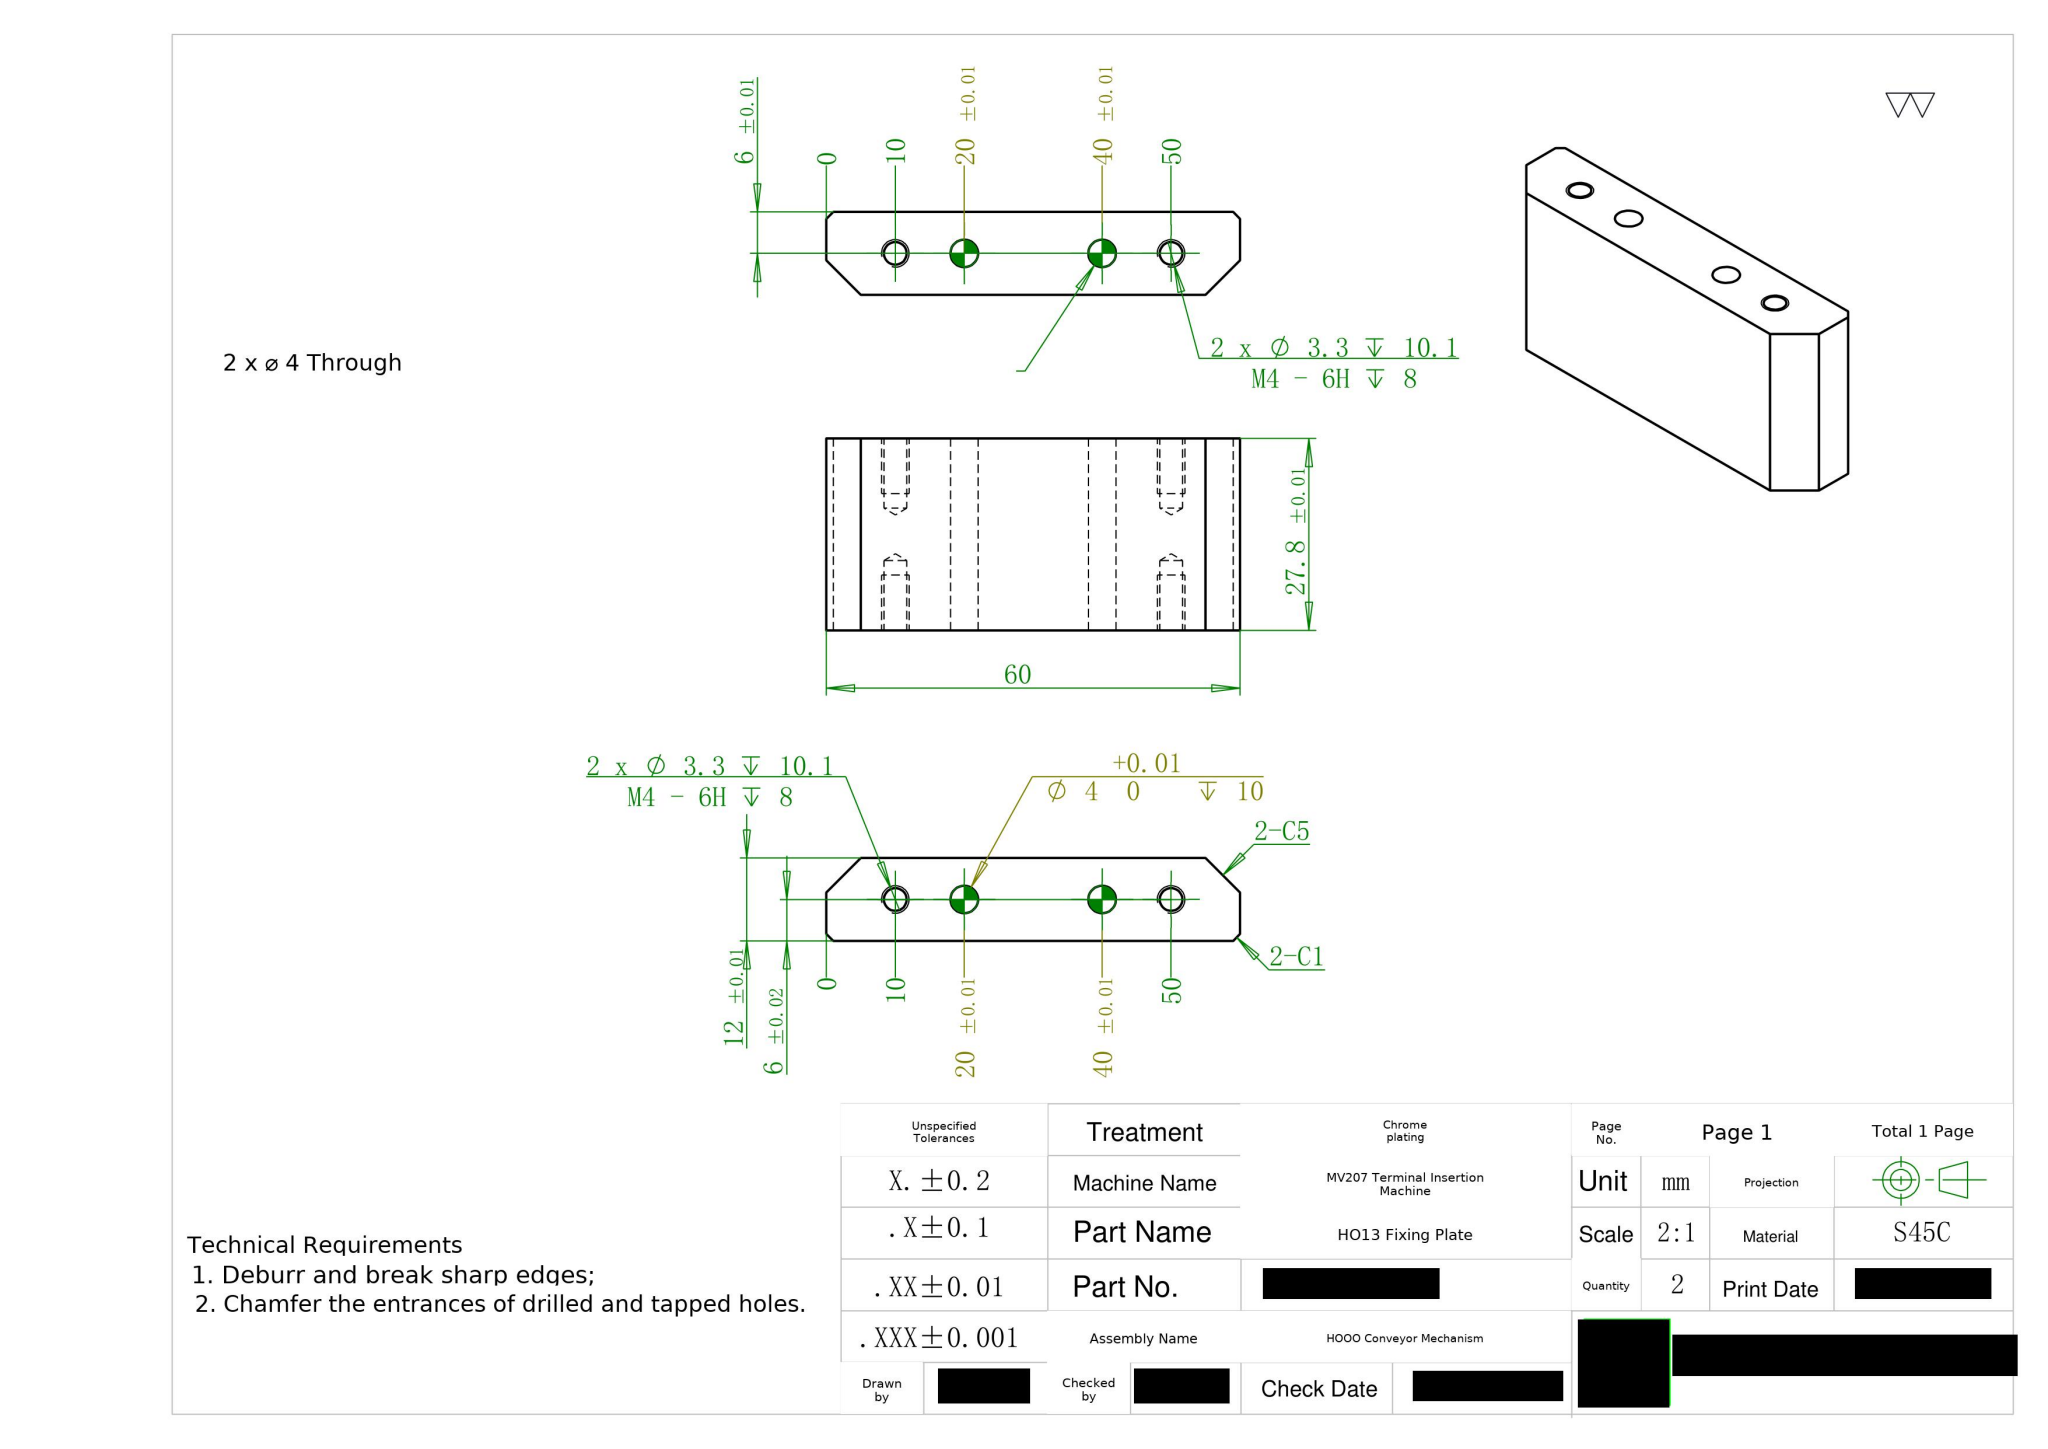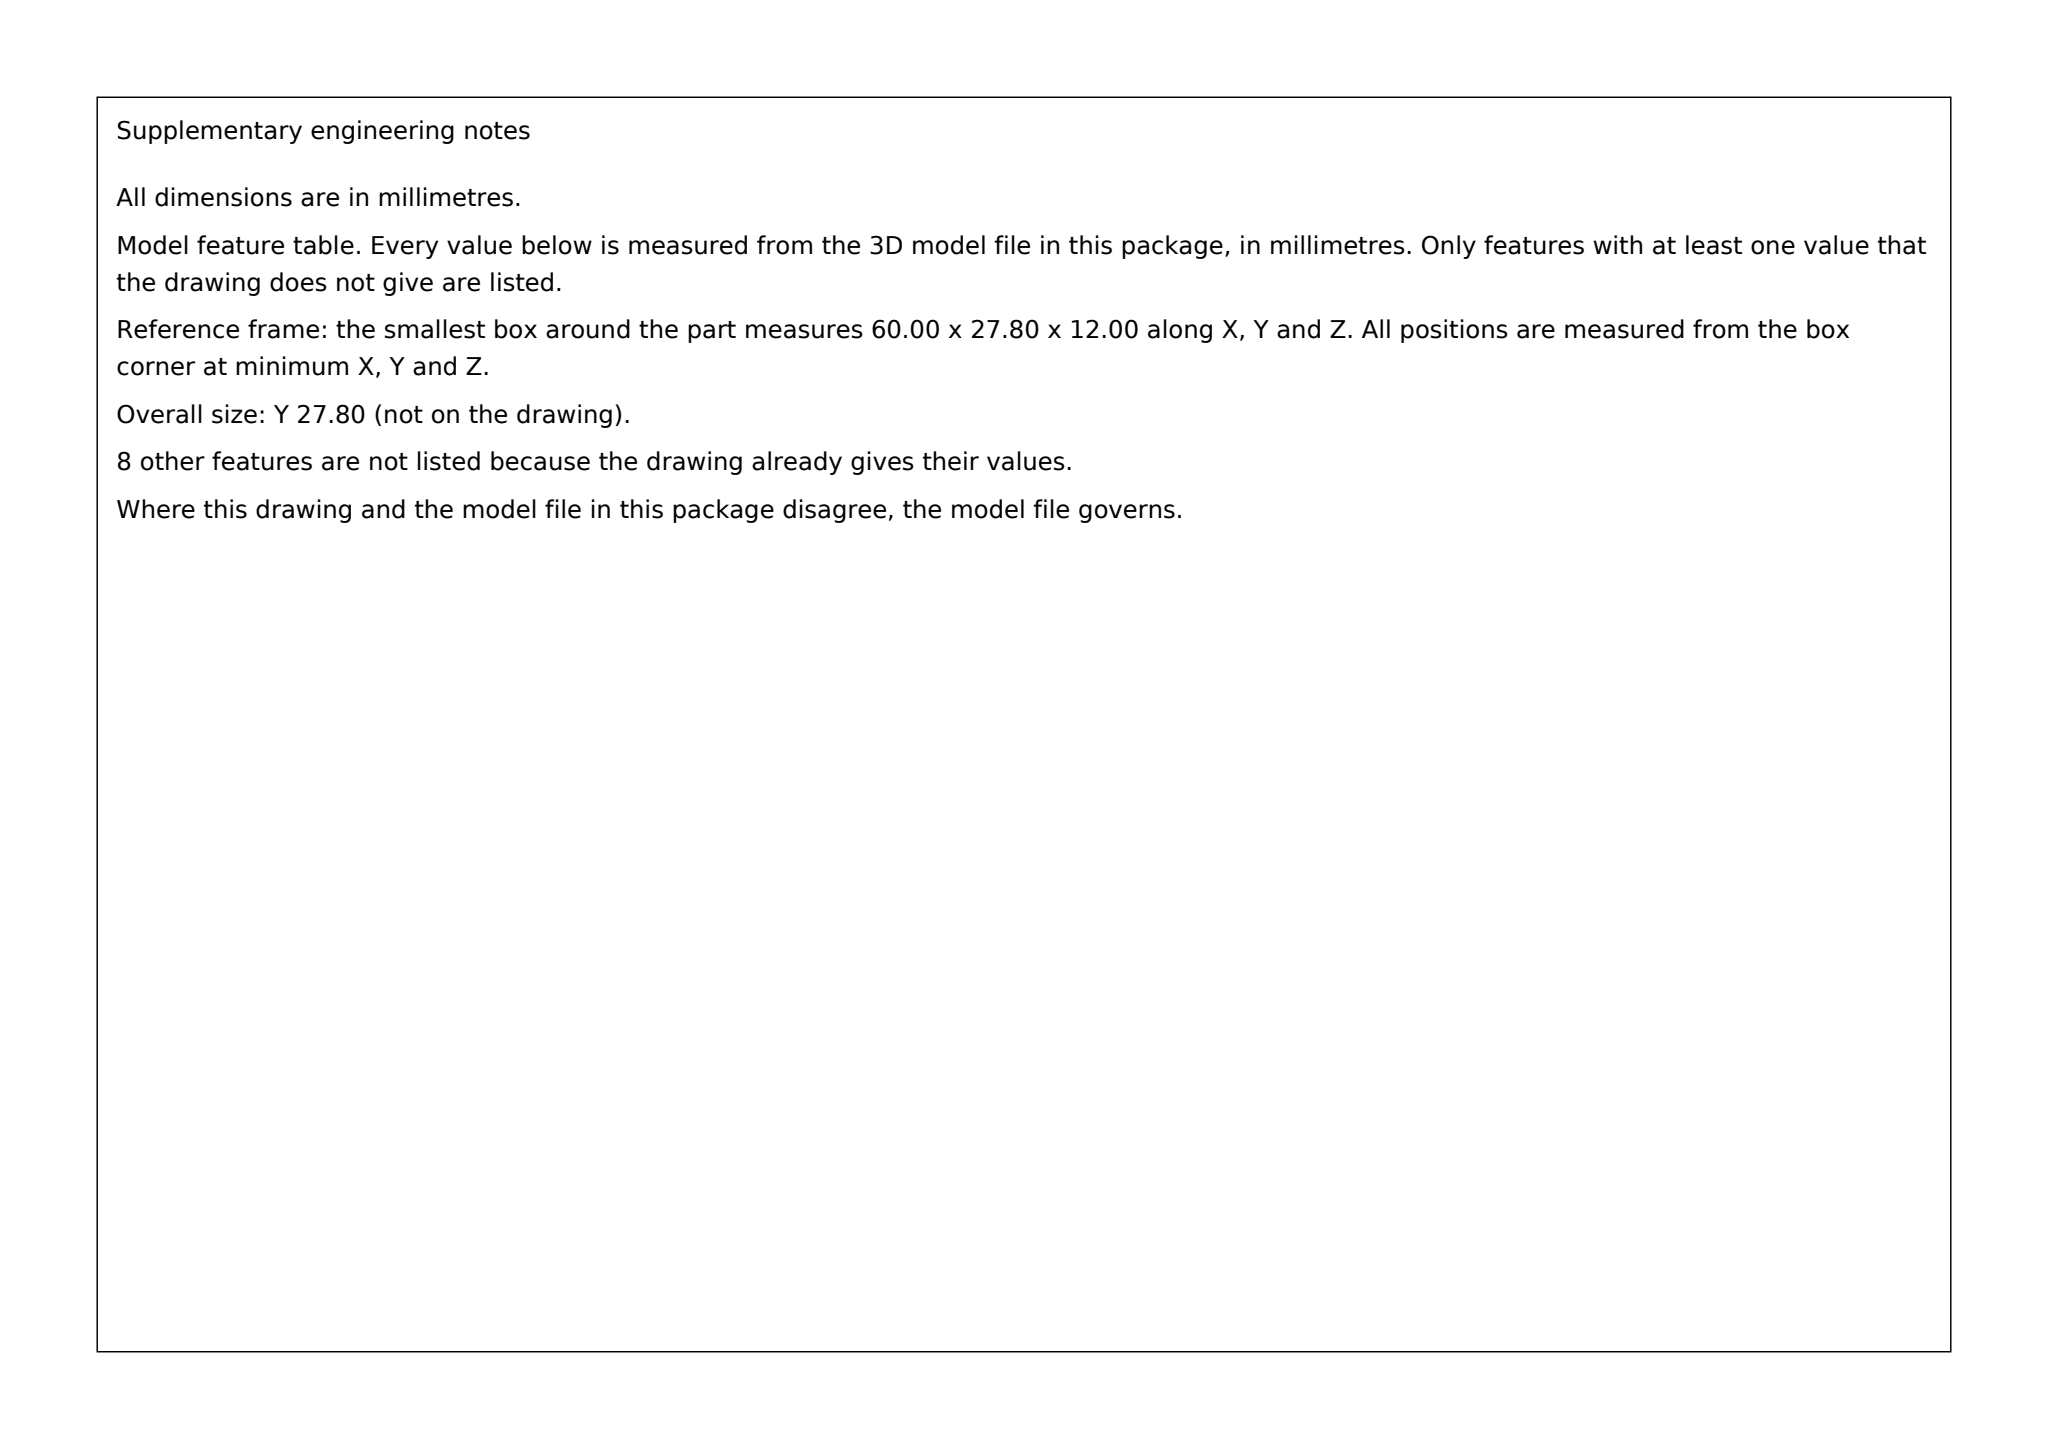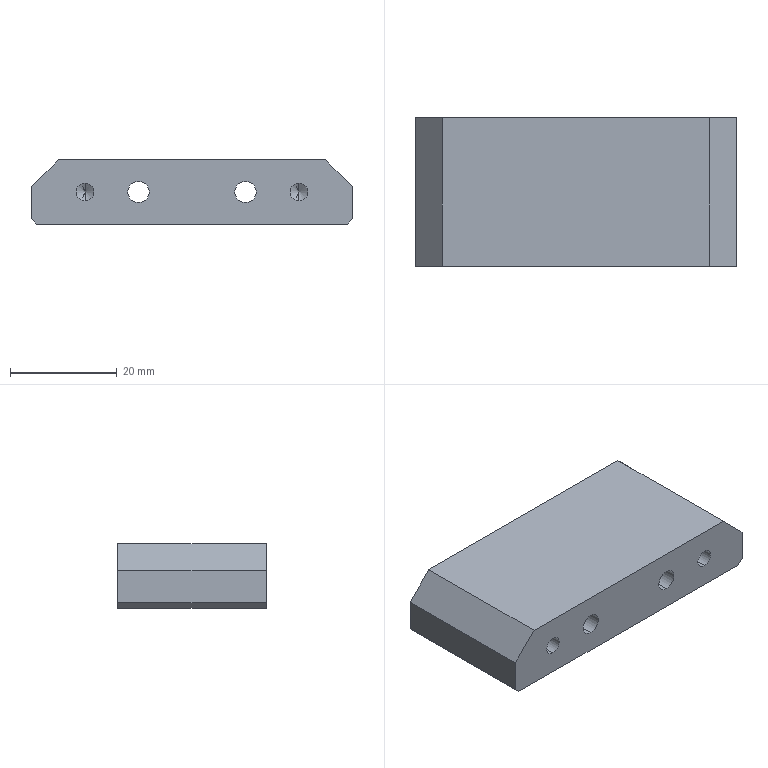Part | SolidWorks | mm | material S45C | 1 solid | 30 faces | box 60 x 27.8 x 12 mm | volume 18238 mm3 | cylinder 12 | plane 10 | cone 8 | commonest cylinder face diameters 3.3 x8 4 x4
build123d program:
from build123d import *

# Parameters (mm, degrees)
SKETCH1_W                    = 60
SKETCH1_H                    = 27.8
BOSS_EXTRUDE1_DEPTH          = 12
M4_TAPPED_HOLE1_D            = 3.3
M4_TAPPED_HOLE1_DEPTH        = 10.1
M4_TAPPED_HOLE1_TIP          = 0.9914
M4_TAPPED_HOLE2_D            = 3.3
M4_TAPPED_HOLE2_DEPTH        = 10.1
M4_TAPPED_HOLE2_TIP          = 0.9914
CHAMFER1_SIZE                = 5
F_4_0_4_DIAMETER_HOLE1_D     = 4
F_4_0_4_DIAMETER_HOLE2_D     = 4
F_4_0_4_DIAMETER_HOLE2_DEPTH = 10
F_4_0_4_DIAMETER_HOLE2_TIP   = 1.202
CHAMFER2_SIZE                = 1


with BuildPart() as part:
    # Sketch1 → Boss-Extrude1 (new body)
    with BuildSketch(Plane.XY):
        Rectangle(SKETCH1_W, SKETCH1_H)
    extrude(amount=BOSS_EXTRUDE1_DEPTH)

    # M4 Tapped Hole1
    with Locations(Plane(origin=(0, 13.9, 0), x_dir=(1, 0, 0), z_dir=(0, 1, 0))):
        with Locations((-20, -6), (20, -6)):
            Hole(M4_TAPPED_HOLE1_D / 2, depth=M4_TAPPED_HOLE1_DEPTH)
            with Locations((0, 0, -(M4_TAPPED_HOLE1_DEPTH + M4_TAPPED_HOLE1_TIP / 2))):  # 118° drill point
                Cone(0, M4_TAPPED_HOLE1_D / 2, M4_TAPPED_HOLE1_TIP, mode=Mode.SUBTRACT)

    # M4 Tapped Hole2
    with Locations(Plane(origin=(0, -13.9, 0), x_dir=(-1, 0, 0), z_dir=(0, -1, 0))):
        with Locations((20, -6), (-20, -6)):
            Hole(M4_TAPPED_HOLE2_D / 2, depth=M4_TAPPED_HOLE2_DEPTH)
            with Locations((0, 0, -(M4_TAPPED_HOLE2_DEPTH + M4_TAPPED_HOLE2_TIP / 2))):  # 118° drill point
                Cone(0, M4_TAPPED_HOLE2_D / 2, M4_TAPPED_HOLE2_TIP, mode=Mode.SUBTRACT)

    # Chamfer1
    chamfer1_edges = [part.edges().sort_by_distance(p)[0] for p in [
        (-30, 0, 12),
        (30, 0, 12),
    ]]
    chamfer(chamfer1_edges, length=CHAMFER1_SIZE)

    # 4.0 _4_ Diameter Hole1 (through all)
    with Locations(Plane(origin=(0, 13.9, 0), x_dir=(1, 0, 0), z_dir=(0, 1, 0))):
        with Locations((-10, -6), (10, -6)):
            Hole(F_4_0_4_DIAMETER_HOLE1_D / 2)

    # 4.0 _4_ Diameter Hole2
    with Locations(Plane(origin=(0, -13.9, 0), x_dir=(-1, 0, 0), z_dir=(0, -1, 0))):
        with Locations((10, -6), (-10, -6)):
            Hole(F_4_0_4_DIAMETER_HOLE2_D / 2, depth=F_4_0_4_DIAMETER_HOLE2_DEPTH)
            with Locations((0, 0, -(F_4_0_4_DIAMETER_HOLE2_DEPTH + F_4_0_4_DIAMETER_HOLE2_TIP / 2))):  # 118° drill point
                Cone(0, F_4_0_4_DIAMETER_HOLE2_D / 2, F_4_0_4_DIAMETER_HOLE2_TIP, mode=Mode.SUBTRACT)

    # Chamfer2
    chamfer2_edges = [part.edges().sort_by_distance(p)[0] for p in [
        (-30, 0, 0),
        (30, 0, 0),
    ]]
    chamfer(chamfer2_edges, length=CHAMFER2_SIZE)


solid = part.part
STEP:
#1=CARTESIAN_POINT('',(-10.,-13.9,4.));
#2=VERTEX_POINT('',#1);
#3=CARTESIAN_POINT('',(-10.,-13.9,8.));
#4=VERTEX_POINT('',#3);
#5=CARTESIAN_POINT('',(-10.,-13.9,6.));
#6=DIRECTION('',(0.,1.,0.));
#7=DIRECTION('',(0.,0.,1.));
#8=AXIS2_PLACEMENT_3D('',#5,#6,#7);
#9=CIRCLE('',#8,2.);
#10=EDGE_CURVE('',#2,#4,#9,.T.);
#11=ORIENTED_EDGE('',*,*,#10,.F.);
#12=CARTESIAN_POINT('',(-10.,13.9,4.));
#13=VERTEX_POINT('',#12);
#14=CARTESIAN_POINT('',(-10.,13.9,4.));
#15=DIRECTION('',(0.,1.,0.));
#16=VECTOR('',#15,1000.);
#17=LINE('',#14,#16);
#18=EDGE_CURVE('',#2,#13,#17,.T.);
#19=ORIENTED_EDGE('',*,*,#18,.T.);
#20=CARTESIAN_POINT('',(-10.,13.9,8.));
#21=VERTEX_POINT('',#20);
#22=CARTESIAN_POINT('',(-10.,13.9,6.));
#23=DIRECTION('',(0.,1.,0.));
#24=DIRECTION('',(0.,0.,1.));
#25=AXIS2_PLACEMENT_3D('',#22,#23,#24);
#26=CIRCLE('',#25,2.);
#27=EDGE_CURVE('',#13,#21,#26,.T.);
#28=ORIENTED_EDGE('',*,*,#27,.T.);
#29=CARTESIAN_POINT('',(-10.,13.9,8.));
#30=DIRECTION('',(0.,1.,0.));
#31=VECTOR('',#30,1000.);
#32=LINE('',#29,#31);
#33=EDGE_CURVE('',#4,#21,#32,.T.);
#34=ORIENTED_EDGE('',*,*,#33,.F.);
#35=EDGE_LOOP('',(#11,#19,#28,#34));
#36=FACE_OUTER_BOUND('',#35,.T.);
#37=CARTESIAN_POINT('',(-10.,13.9,6.));
#38=DIRECTION('',(0.,1.,0.));
#39=DIRECTION('',(0.,0.,1.));
#40=AXIS2_PLACEMENT_3D('',#37,#38,#39);
#41=CYLINDRICAL_SURFACE('',#40,2.);
#42=ADVANCED_FACE('',(#36),#41,.F.);
#43=CARTESIAN_POINT('',(10.,-13.9,4.));
#44=VERTEX_POINT('',#43);
#45=CARTESIAN_POINT('',(10.,-13.9,8.));
#46=VERTEX_POINT('',#45);
#47=CARTESIAN_POINT('',(10.,-13.9,6.));
#48=DIRECTION('',(0.,1.,0.));
#49=DIRECTION('',(0.,0.,1.));
#50=AXIS2_PLACEMENT_3D('',#47,#48,#49);
#51=CIRCLE('',#50,2.);
#52=EDGE_CURVE('',#44,#46,#51,.T.);
#53=ORIENTED_EDGE('',*,*,#52,.F.);
#54=CARTESIAN_POINT('',(10.,13.9,4.));
#55=VERTEX_POINT('',#54);
#56=CARTESIAN_POINT('',(10.,13.9,4.));
#57=DIRECTION('',(0.,1.,0.));
#58=VECTOR('',#57,1000.);
#59=LINE('',#56,#58);
#60=EDGE_CURVE('',#44,#55,#59,.T.);
#61=ORIENTED_EDGE('',*,*,#60,.T.);
#62=CARTESIAN_POINT('',(10.,13.9,8.));
#63=VERTEX_POINT('',#62);
#64=CARTESIAN_POINT('',(10.,13.9,6.));
#65=DIRECTION('',(0.,1.,0.));
#66=DIRECTION('',(0.,0.,1.));
#67=AXIS2_PLACEMENT_3D('',#64,#65,#66);
#68=CIRCLE('',#67,2.);
#69=EDGE_CURVE('',#55,#63,#68,.T.);
#70=ORIENTED_EDGE('',*,*,#69,.T.);
#71=CARTESIAN_POINT('',(10.,13.9,8.));
#72=DIRECTION('',(0.,1.,0.));
#73=VECTOR('',#72,1000.);
#74=LINE('',#71,#73);
#75=EDGE_CURVE('',#46,#63,#74,.T.);
#76=ORIENTED_EDGE('',*,*,#75,.F.);
#77=EDGE_LOOP('',(#53,#61,#70,#76));
#78=FACE_OUTER_BOUND('',#77,.T.);
#79=CARTESIAN_POINT('',(10.,13.9,6.));
#80=DIRECTION('',(0.,1.,0.));
#81=DIRECTION('',(0.,0.,1.));
#82=AXIS2_PLACEMENT_3D('',#79,#80,#81);
#83=CYLINDRICAL_SURFACE('',#82,2.);
#84=ADVANCED_FACE('',(#78),#83,.F.);
#85=CARTESIAN_POINT('',(-20.,-3.8,7.65));
#86=VERTEX_POINT('',#85);
#87=CARTESIAN_POINT('',(-20.,-3.8,4.35));
#88=VERTEX_POINT('',#87);
#89=CARTESIAN_POINT('',(-20.,-3.8,6.));
#90=DIRECTION('',(0.,-1.,0.));
#91=DIRECTION('',(0.,0.,-1.));
#92=AXIS2_PLACEMENT_3D('',#89,#90,#91);
#93=CIRCLE('',#92,1.65);
#94=EDGE_CURVE('',#86,#88,#93,.T.);
#95=ORIENTED_EDGE('',*,*,#94,.F.);
#96=CARTESIAN_POINT('',(-20.,-13.9,7.65));
#97=VERTEX_POINT('',#96);
#98=CARTESIAN_POINT('',(-20.,-13.9,7.65));
#99=DIRECTION('',(0.,-1.,0.));
#100=VECTOR('',#99,1000.);
#101=LINE('',#98,#100);
#102=EDGE_CURVE('',#86,#97,#101,.T.);
#103=ORIENTED_EDGE('',*,*,#102,.T.);
#104=CARTESIAN_POINT('',(-20.,-13.9,4.35));
#105=VERTEX_POINT('',#104);
#106=CARTESIAN_POINT('',(-20.,-13.9,6.));
#107=DIRECTION('',(0.,-1.,0.));
#108=DIRECTION('',(0.,0.,-1.));
#109=AXIS2_PLACEMENT_3D('',#106,#107,#108);
#110=CIRCLE('',#109,1.65);
#111=EDGE_CURVE('',#97,#105,#110,.T.);
#112=ORIENTED_EDGE('',*,*,#111,.T.);
#113=CARTESIAN_POINT('',(-20.,-13.9,4.35));
#114=DIRECTION('',(0.,-1.,0.));
#115=VECTOR('',#114,1000.);
#116=LINE('',#113,#115);
#117=EDGE_CURVE('',#88,#105,#116,.T.);
#118=ORIENTED_EDGE('',*,*,#117,.F.);
#119=EDGE_LOOP('',(#95,#103,#112,#118));
#120=FACE_OUTER_BOUND('',#119,.T.);
#121=CARTESIAN_POINT('',(-20.,-13.9,6.));
#122=DIRECTION('',(0.,-1.,0.));
#123=DIRECTION('',(0.,0.,-1.));
#124=AXIS2_PLACEMENT_3D('',#121,#122,#123);
#125=CYLINDRICAL_SURFACE('',#124,1.65);
#126=ADVANCED_FACE('',(#120),#125,.F.);
#127=CARTESIAN_POINT('',(-20.,-2.809,6.));
#128=VERTEX_POINT('',#127);
#129=CARTESIAN_POINT('',(-20.,-3.8,4.35));
#130=DIRECTION('',(0.,-0.515,-0.8572));
#131=VECTOR('',#130,1000.);
#132=LINE('',#129,#131);
#133=EDGE_CURVE('',#128,#88,#132,.T.);
#134=ORIENTED_EDGE('',*,*,#133,.F.);
#135=CARTESIAN_POINT('',(-20.,-3.8,7.65));
#136=DIRECTION('',(0.,-0.515,0.8572));
#137=VECTOR('',#136,1000.);
#138=LINE('',#135,#137);
#139=EDGE_CURVE('',#128,#86,#138,.T.);
#140=ORIENTED_EDGE('',*,*,#139,.T.);
#141=ORIENTED_EDGE('',*,*,#94,.T.);
#142=EDGE_LOOP('',(#134,#140,#141));
#143=FACE_OUTER_BOUND('',#142,.T.);
#144=CARTESIAN_POINT('',(-20.,-3.8,6.));
#145=DIRECTION('',(0.,-1.,0.));
#146=DIRECTION('',(0.,0.,-1.));
#147=AXIS2_PLACEMENT_3D('',#144,#145,#146);
#148=CONICAL_SURFACE('',#147,1.65,1.03);
#149=ADVANCED_FACE('',(#143),#148,.F.);
#150=CARTESIAN_POINT('',(20.,-3.8,7.65));
#151=VERTEX_POINT('',#150);
#152=CARTESIAN_POINT('',(20.,-3.8,4.35));
#153=VERTEX_POINT('',#152);
#154=CARTESIAN_POINT('',(20.,-3.8,6.));
#155=DIRECTION('',(0.,-1.,0.));
#156=DIRECTION('',(0.,0.,-1.));
#157=AXIS2_PLACEMENT_3D('',#154,#155,#156);
#158=CIRCLE('',#157,1.65);
#159=EDGE_CURVE('',#151,#153,#158,.T.);
#160=ORIENTED_EDGE('',*,*,#159,.F.);
#161=CARTESIAN_POINT('',(20.,-13.9,7.65));
#162=VERTEX_POINT('',#161);
#163=CARTESIAN_POINT('',(20.,-13.9,7.65));
#164=DIRECTION('',(0.,-1.,0.));
#165=VECTOR('',#164,1000.);
#166=LINE('',#163,#165);
#167=EDGE_CURVE('',#151,#162,#166,.T.);
#168=ORIENTED_EDGE('',*,*,#167,.T.);
#169=CARTESIAN_POINT('',(20.,-13.9,4.35));
#170=VERTEX_POINT('',#169);
#171=CARTESIAN_POINT('',(20.,-13.9,6.));
#172=DIRECTION('',(0.,-1.,0.));
#173=DIRECTION('',(0.,0.,-1.));
#174=AXIS2_PLACEMENT_3D('',#171,#172,#173);
#175=CIRCLE('',#174,1.65);
#176=EDGE_CURVE('',#162,#170,#175,.T.);
#177=ORIENTED_EDGE('',*,*,#176,.T.);
#178=CARTESIAN_POINT('',(20.,-13.9,4.35));
#179=DIRECTION('',(0.,-1.,0.));
#180=VECTOR('',#179,1000.);
#181=LINE('',#178,#180);
#182=EDGE_CURVE('',#153,#170,#181,.T.);
#183=ORIENTED_EDGE('',*,*,#182,.F.);
#184=EDGE_LOOP('',(#160,#168,#177,#183));
#185=FACE_OUTER_BOUND('',#184,.T.);
#186=CARTESIAN_POINT('',(20.,-13.9,6.));
#187=DIRECTION('',(0.,-1.,0.));
#188=DIRECTION('',(0.,0.,-1.));
#189=AXIS2_PLACEMENT_3D('',#186,#187,#188);
#190=CYLINDRICAL_SURFACE('',#189,1.65);
#191=ADVANCED_FACE('',(#185),#190,.F.);
#192=CARTESIAN_POINT('',(20.,-2.809,6.));
#193=VERTEX_POINT('',#192);
#194=CARTESIAN_POINT('',(20.,-3.8,4.35));
#195=DIRECTION('',(0.,-0.515,-0.8572));
#196=VECTOR('',#195,1000.);
#197=LINE('',#194,#196);
#198=EDGE_CURVE('',#193,#153,#197,.T.);
#199=ORIENTED_EDGE('',*,*,#198,.F.);
#200=CARTESIAN_POINT('',(20.,-3.8,7.65));
#201=DIRECTION('',(0.,-0.515,0.8572));
#202=VECTOR('',#201,1000.);
#203=LINE('',#200,#202);
#204=EDGE_CURVE('',#193,#151,#203,.T.);
#205=ORIENTED_EDGE('',*,*,#204,.T.);
#206=ORIENTED_EDGE('',*,*,#159,.T.);
#207=EDGE_LOOP('',(#199,#205,#206));
#208=FACE_OUTER_BOUND('',#207,.T.);
#209=CARTESIAN_POINT('',(20.,-3.8,6.));
#210=DIRECTION('',(0.,-1.,0.));
#211=DIRECTION('',(0.,0.,-1.));
#212=AXIS2_PLACEMENT_3D('',#209,#210,#211);
#213=CONICAL_SURFACE('',#212,1.65,1.03);
#214=ADVANCED_FACE('',(#208),#213,.F.);
#215=CARTESIAN_POINT('',(-20.,3.8,4.35));
#216=VERTEX_POINT('',#215);
#217=CARTESIAN_POINT('',(-20.,3.8,7.65));
#218=VERTEX_POINT('',#217);
#219=CARTESIAN_POINT('',(-20.,3.8,6.));
#220=DIRECTION('',(0.,1.,0.));
#221=DIRECTION('',(0.,0.,1.));
#222=AXIS2_PLACEMENT_3D('',#219,#220,#221);
#223=CIRCLE('',#222,1.65);
#224=EDGE_CURVE('',#216,#218,#223,.T.);
#225=ORIENTED_EDGE('',*,*,#224,.F.);
#226=CARTESIAN_POINT('',(-20.,13.9,4.35));
#227=VERTEX_POINT('',#226);
#228=CARTESIAN_POINT('',(-20.,13.9,4.35));
#229=DIRECTION('',(0.,1.,0.));
#230=VECTOR('',#229,1000.);
#231=LINE('',#228,#230);
#232=EDGE_CURVE('',#216,#227,#231,.T.);
#233=ORIENTED_EDGE('',*,*,#232,.T.);
#234=CARTESIAN_POINT('',(-20.,13.9,7.65));
#235=VERTEX_POINT('',#234);
#236=CARTESIAN_POINT('',(-20.,13.9,6.));
#237=DIRECTION('',(0.,1.,0.));
#238=DIRECTION('',(0.,0.,1.));
#239=AXIS2_PLACEMENT_3D('',#236,#237,#238);
#240=CIRCLE('',#239,1.65);
#241=EDGE_CURVE('',#227,#235,#240,.T.);
#242=ORIENTED_EDGE('',*,*,#241,.T.);
#243=CARTESIAN_POINT('',(-20.,13.9,7.65));
#244=DIRECTION('',(0.,1.,0.));
#245=VECTOR('',#244,1000.);
#246=LINE('',#243,#245);
#247=EDGE_CURVE('',#218,#235,#246,.T.);
#248=ORIENTED_EDGE('',*,*,#247,.F.);
#249=EDGE_LOOP('',(#225,#233,#242,#248));
#250=FACE_OUTER_BOUND('',#249,.T.);
#251=CARTESIAN_POINT('',(-20.,13.9,6.));
#252=DIRECTION('',(0.,1.,0.));
#253=DIRECTION('',(0.,0.,1.));
#254=AXIS2_PLACEMENT_3D('',#251,#252,#253);
#255=CYLINDRICAL_SURFACE('',#254,1.65);
#256=ADVANCED_FACE('',(#250),#255,.F.);
#257=CARTESIAN_POINT('',(-20.,2.809,6.));
#258=VERTEX_POINT('',#257);
#259=CARTESIAN_POINT('',(-20.,3.8,7.65));
#260=DIRECTION('',(0.,0.515,0.8572));
#261=VECTOR('',#260,1000.);
#262=LINE('',#259,#261);
#263=EDGE_CURVE('',#258,#218,#262,.T.);
#264=ORIENTED_EDGE('',*,*,#263,.F.);
#265=CARTESIAN_POINT('',(-20.,3.8,4.35));
#266=DIRECTION('',(0.,0.515,-0.8572));
#267=VECTOR('',#266,1000.);
#268=LINE('',#265,#267);
#269=EDGE_CURVE('',#258,#216,#268,.T.);
#270=ORIENTED_EDGE('',*,*,#269,.T.);
#271=ORIENTED_EDGE('',*,*,#224,.T.);
#272=EDGE_LOOP('',(#264,#270,#271));
#273=FACE_OUTER_BOUND('',#272,.T.);
#274=CARTESIAN_POINT('',(-20.,3.8,6.));
#275=DIRECTION('',(0.,1.,0.));
#276=DIRECTION('',(0.,0.,1.));
#277=AXIS2_PLACEMENT_3D('',#274,#275,#276);
#278=CONICAL_SURFACE('',#277,1.65,1.03);
#279=ADVANCED_FACE('',(#273),#278,.F.);
#280=CARTESIAN_POINT('',(20.,3.8,4.35));
#281=VERTEX_POINT('',#280);
#282=CARTESIAN_POINT('',(20.,3.8,7.65));
#283=VERTEX_POINT('',#282);
#284=CARTESIAN_POINT('',(20.,3.8,6.));
#285=DIRECTION('',(0.,1.,0.));
#286=DIRECTION('',(0.,0.,1.));
#287=AXIS2_PLACEMENT_3D('',#284,#285,#286);
#288=CIRCLE('',#287,1.65);
#289=EDGE_CURVE('',#281,#283,#288,.T.);
#290=ORIENTED_EDGE('',*,*,#289,.F.);
#291=CARTESIAN_POINT('',(20.,13.9,4.35));
#292=VERTEX_POINT('',#291);
#293=CARTESIAN_POINT('',(20.,13.9,4.35));
#294=DIRECTION('',(0.,1.,0.));
#295=VECTOR('',#294,1000.);
#296=LINE('',#293,#295);
#297=EDGE_CURVE('',#281,#292,#296,.T.);
#298=ORIENTED_EDGE('',*,*,#297,.T.);
#299=CARTESIAN_POINT('',(20.,13.9,7.65));
#300=VERTEX_POINT('',#299);
#301=CARTESIAN_POINT('',(20.,13.9,6.));
#302=DIRECTION('',(0.,1.,0.));
#303=DIRECTION('',(0.,0.,1.));
#304=AXIS2_PLACEMENT_3D('',#301,#302,#303);
#305=CIRCLE('',#304,1.65);
#306=EDGE_CURVE('',#292,#300,#305,.T.);
#307=ORIENTED_EDGE('',*,*,#306,.T.);
#308=CARTESIAN_POINT('',(20.,13.9,7.65));
#309=DIRECTION('',(0.,1.,0.));
#310=VECTOR('',#309,1000.);
#311=LINE('',#308,#310);
#312=EDGE_CURVE('',#283,#300,#311,.T.);
#313=ORIENTED_EDGE('',*,*,#312,.F.);
#314=EDGE_LOOP('',(#290,#298,#307,#313));
#315=FACE_OUTER_BOUND('',#314,.T.);
#316=CARTESIAN_POINT('',(20.,13.9,6.));
#317=DIRECTION('',(0.,1.,0.));
#318=DIRECTION('',(0.,0.,1.));
#319=AXIS2_PLACEMENT_3D('',#316,#317,#318);
#320=CYLINDRICAL_SURFACE('',#319,1.65);
#321=ADVANCED_FACE('',(#315),#320,.F.);
#322=CARTESIAN_POINT('',(20.,2.809,6.));
#323=VERTEX_POINT('',#322);
#324=CARTESIAN_POINT('',(20.,3.8,7.65));
#325=DIRECTION('',(0.,0.515,0.8572));
#326=VECTOR('',#325,1000.);
#327=LINE('',#324,#326);
#328=EDGE_CURVE('',#323,#283,#327,.T.);
#329=ORIENTED_EDGE('',*,*,#328,.F.);
#330=CARTESIAN_POINT('',(20.,3.8,4.35));
#331=DIRECTION('',(0.,0.515,-0.8572));
#332=VECTOR('',#331,1000.);
#333=LINE('',#330,#332);
#334=EDGE_CURVE('',#323,#281,#333,.T.);
#335=ORIENTED_EDGE('',*,*,#334,.T.);
#336=ORIENTED_EDGE('',*,*,#289,.T.);
#337=EDGE_LOOP('',(#329,#335,#336));
#338=FACE_OUTER_BOUND('',#337,.T.);
#339=CARTESIAN_POINT('',(20.,3.8,6.));
#340=DIRECTION('',(0.,1.,0.));
#341=DIRECTION('',(0.,0.,1.));
#342=AXIS2_PLACEMENT_3D('',#339,#340,#341);
#343=CONICAL_SURFACE('',#342,1.65,1.03);
#344=ADVANCED_FACE('',(#338),#343,.F.);
#345=CARTESIAN_POINT('',(30.,-13.9,7.));
#346=VERTEX_POINT('',#345);
#347=CARTESIAN_POINT('',(30.,-13.9,1.));
#348=VERTEX_POINT('',#347);
#349=CARTESIAN_POINT('',(30.,-13.9,12.));
#350=DIRECTION('',(0.,0.,-1.));
#351=VECTOR('',#350,1000.);
#352=LINE('',#349,#351);
#353=EDGE_CURVE('',#346,#348,#352,.T.);
#354=ORIENTED_EDGE('',*,*,#353,.T.);
#355=CARTESIAN_POINT('',(30.,13.9,1.));
#356=VERTEX_POINT('',#355);
#357=CARTESIAN_POINT('',(30.,13.9,1.));
#358=DIRECTION('',(0.,1.,0.));
#359=VECTOR('',#358,1000.);
#360=LINE('',#357,#359);
#361=EDGE_CURVE('',#348,#356,#360,.T.);
#362=ORIENTED_EDGE('',*,*,#361,.T.);
#363=CARTESIAN_POINT('',(30.,13.9,7.));
#364=VERTEX_POINT('',#363);
#365=CARTESIAN_POINT('',(30.,13.9,12.));
#366=DIRECTION('',(0.,0.,-1.));
#367=VECTOR('',#366,1000.);
#368=LINE('',#365,#367);
#369=EDGE_CURVE('',#364,#356,#368,.T.);
#370=ORIENTED_EDGE('',*,*,#369,.F.);
#371=CARTESIAN_POINT('',(30.,-13.9,7.));
#372=DIRECTION('',(0.,-1.,0.));
#373=VECTOR('',#372,1000.);
#374=LINE('',#371,#373);
#375=EDGE_CURVE('',#364,#346,#374,.T.);
#376=ORIENTED_EDGE('',*,*,#375,.T.);
#377=EDGE_LOOP('',(#354,#362,#370,#376));
#378=FACE_OUTER_BOUND('',#377,.T.);
#379=CARTESIAN_POINT('',(30.,13.9,12.));
#380=DIRECTION('',(-1.,0.,0.));
#381=DIRECTION('',(0.,0.,1.));
#382=AXIS2_PLACEMENT_3D('',#379,#380,#381);
#383=PLANE('',#382);
#384=ADVANCED_FACE('',(#378),#383,.F.);
#385=CARTESIAN_POINT('',(-10.,13.9,6.));
#386=DIRECTION('',(0.,1.,0.));
#387=DIRECTION('',(0.,0.,1.));
#388=AXIS2_PLACEMENT_3D('',#385,#386,#387);
#389=CIRCLE('',#388,2.);
#390=EDGE_CURVE('',#21,#13,#389,.T.);
#391=ORIENTED_EDGE('',*,*,#390,.F.);
#392=ORIENTED_EDGE('',*,*,#27,.F.);
#393=EDGE_LOOP('',(#391,#392));
#394=FACE_BOUND('',#393,.T.);
#395=CARTESIAN_POINT('',(10.,13.9,6.));
#396=DIRECTION('',(0.,1.,0.));
#397=DIRECTION('',(0.,0.,1.));
#398=AXIS2_PLACEMENT_3D('',#395,#396,#397);
#399=CIRCLE('',#398,2.);
#400=EDGE_CURVE('',#63,#55,#399,.T.);
#401=ORIENTED_EDGE('',*,*,#400,.F.);
#402=ORIENTED_EDGE('',*,*,#69,.F.);
#403=EDGE_LOOP('',(#401,#402));
#404=FACE_BOUND('',#403,.T.);
#405=CARTESIAN_POINT('',(-20.,13.9,6.));
#406=DIRECTION('',(0.,1.,0.));
#407=DIRECTION('',(0.,0.,1.));
#408=AXIS2_PLACEMENT_3D('',#405,#406,#407);
#409=CIRCLE('',#408,1.65);
#410=EDGE_CURVE('',#235,#227,#409,.T.);
#411=ORIENTED_EDGE('',*,*,#410,.F.);
#412=ORIENTED_EDGE('',*,*,#241,.F.);
#413=EDGE_LOOP('',(#411,#412));
#414=FACE_BOUND('',#413,.T.);
#415=CARTESIAN_POINT('',(20.,13.9,6.));
#416=DIRECTION('',(0.,1.,0.));
#417=DIRECTION('',(0.,0.,1.));
#418=AXIS2_PLACEMENT_3D('',#415,#416,#417);
#419=CIRCLE('',#418,1.65);
#420=EDGE_CURVE('',#300,#292,#419,.T.);
#421=ORIENTED_EDGE('',*,*,#420,.F.);
#422=ORIENTED_EDGE('',*,*,#306,.F.);
#423=EDGE_LOOP('',(#421,#422));
#424=FACE_BOUND('',#423,.T.);
#425=CARTESIAN_POINT('',(29.,13.9,0.));
#426=VERTEX_POINT('',#425);
#427=CARTESIAN_POINT('',(-29.,13.9,0.));
#428=VERTEX_POINT('',#427);
#429=CARTESIAN_POINT('',(-30.,13.9,0.));
#430=DIRECTION('',(-1.,0.,0.));
#431=VECTOR('',#430,1000.);
#432=LINE('',#429,#431);
#433=EDGE_CURVE('',#426,#428,#432,.T.);
#434=ORIENTED_EDGE('',*,*,#433,.T.);
#435=CARTESIAN_POINT('',(-30.,13.9,1.));
#436=VERTEX_POINT('',#435);
#437=CARTESIAN_POINT('',(-30.,13.9,1.));
#438=DIRECTION('',(-0.7071,0.,0.7071));
#439=VECTOR('',#438,1000.);
#440=LINE('',#437,#439);
#441=EDGE_CURVE('',#428,#436,#440,.T.);
#442=ORIENTED_EDGE('',*,*,#441,.T.);
#443=CARTESIAN_POINT('',(-30.,13.9,7.));
#444=VERTEX_POINT('',#443);
#445=CARTESIAN_POINT('',(-30.,13.9,12.));
#446=DIRECTION('',(0.,0.,-1.));
#447=VECTOR('',#446,1000.);
#448=LINE('',#445,#447);
#449=EDGE_CURVE('',#444,#436,#448,.T.);
#450=ORIENTED_EDGE('',*,*,#449,.F.);
#451=CARTESIAN_POINT('',(-25.,13.9,12.));
#452=VERTEX_POINT('',#451);
#453=CARTESIAN_POINT('',(-25.,13.9,12.));
#454=DIRECTION('',(0.7071,0.,0.7071));
#455=VECTOR('',#454,1000.);
#456=LINE('',#453,#455);
#457=EDGE_CURVE('',#444,#452,#456,.T.);
#458=ORIENTED_EDGE('',*,*,#457,.T.);
#459=CARTESIAN_POINT('',(25.,13.9,12.));
#460=VERTEX_POINT('',#459);
#461=CARTESIAN_POINT('',(-30.,13.9,12.));
#462=DIRECTION('',(-1.,0.,0.));
#463=VECTOR('',#462,1000.);
#464=LINE('',#461,#463);
#465=EDGE_CURVE('',#460,#452,#464,.T.);
#466=ORIENTED_EDGE('',*,*,#465,.F.);
#467=CARTESIAN_POINT('',(25.,13.9,12.));
#468=DIRECTION('',(0.7071,0.,-0.7071));
#469=VECTOR('',#468,1000.);
#470=LINE('',#467,#469);
#471=EDGE_CURVE('',#460,#364,#470,.T.);
#472=ORIENTED_EDGE('',*,*,#471,.T.);
#473=ORIENTED_EDGE('',*,*,#369,.T.);
#474=CARTESIAN_POINT('',(30.,13.9,1.));
#475=DIRECTION('',(-0.7071,0.,-0.7071));
#476=VECTOR('',#475,1000.);
#477=LINE('',#474,#476);
#478=EDGE_CURVE('',#356,#426,#477,.T.);
#479=ORIENTED_EDGE('',*,*,#478,.T.);
#480=EDGE_LOOP('',(#434,#442,#450,#458,#466,#472,#473,#479));
#481=FACE_OUTER_BOUND('',#480,.T.);
#482=CARTESIAN_POINT('',(-30.,13.9,12.));
#483=DIRECTION('',(0.,-1.,0.));
#484=DIRECTION('',(0.,0.,-1.));
#485=AXIS2_PLACEMENT_3D('',#482,#483,#484);
#486=PLANE('',#485);
#487=ADVANCED_FACE('',(#394,#404,#414,#424,#481),#486,.F.);
#488=ORIENTED_EDGE('',*,*,#449,.T.);
#489=CARTESIAN_POINT('',(-30.,-13.9,1.));
#490=VERTEX_POINT('',#489);
#491=CARTESIAN_POINT('',(-30.,13.9,1.));
#492=DIRECTION('',(0.,-1.,0.));
#493=VECTOR('',#492,1000.);
#494=LINE('',#491,#493);
#495=EDGE_CURVE('',#436,#490,#494,.T.);
#496=ORIENTED_EDGE('',*,*,#495,.T.);
#497=CARTESIAN_POINT('',(-30.,-13.9,7.));
#498=VERTEX_POINT('',#497);
#499=CARTESIAN_POINT('',(-30.,-13.9,12.));
#500=DIRECTION('',(0.,0.,-1.));
#501=VECTOR('',#500,1000.);
#502=LINE('',#499,#501);
#503=EDGE_CURVE('',#498,#490,#502,.T.);
#504=ORIENTED_EDGE('',*,*,#503,.F.);
#505=CARTESIAN_POINT('',(-30.,13.9,7.));
#506=DIRECTION('',(0.,1.,0.));
#507=VECTOR('',#506,1000.);
#508=LINE('',#505,#507);
#509=EDGE_CURVE('',#498,#444,#508,.T.);
#510=ORIENTED_EDGE('',*,*,#509,.T.);
#511=EDGE_LOOP('',(#488,#496,#504,#510));
#512=FACE_OUTER_BOUND('',#511,.T.);
#513=CARTESIAN_POINT('',(-30.,13.9,12.));
#514=DIRECTION('',(1.,0.,0.));
#515=DIRECTION('',(0.,0.,-1.));
#516=AXIS2_PLACEMENT_3D('',#513,#514,#515);
#517=PLANE('',#516);
#518=ADVANCED_FACE('',(#512),#517,.F.);
#519=CARTESIAN_POINT('',(-10.,-13.9,6.));
#520=DIRECTION('',(0.,1.,0.));
#521=DIRECTION('',(0.,0.,1.));
#522=AXIS2_PLACEMENT_3D('',#519,#520,#521);
#523=CIRCLE('',#522,2.);
#524=EDGE_CURVE('',#4,#2,#523,.T.);
#525=ORIENTED_EDGE('',*,*,#524,.T.);
#526=ORIENTED_EDGE('',*,*,#10,.T.);
#527=EDGE_LOOP('',(#525,#526));
#528=FACE_BOUND('',#527,.T.);
#529=CARTESIAN_POINT('',(10.,-13.9,6.));
#530=DIRECTION('',(0.,1.,0.));
#531=DIRECTION('',(0.,0.,1.));
#532=AXIS2_PLACEMENT_3D('',#529,#530,#531);
#533=CIRCLE('',#532,2.);
#534=EDGE_CURVE('',#46,#44,#533,.T.);
#535=ORIENTED_EDGE('',*,*,#534,.T.);
#536=ORIENTED_EDGE('',*,*,#52,.T.);
#537=EDGE_LOOP('',(#535,#536));
#538=FACE_BOUND('',#537,.T.);
#539=CARTESIAN_POINT('',(-20.,-13.9,6.));
#540=DIRECTION('',(0.,-1.,0.));
#541=DIRECTION('',(0.,0.,-1.));
#542=AXIS2_PLACEMENT_3D('',#539,#540,#541);
#543=CIRCLE('',#542,1.65);
#544=EDGE_CURVE('',#105,#97,#543,.T.);
#545=ORIENTED_EDGE('',*,*,#544,.F.);
#546=ORIENTED_EDGE('',*,*,#111,.F.);
#547=EDGE_LOOP('',(#545,#546));
#548=FACE_BOUND('',#547,.T.);
#549=CARTESIAN_POINT('',(20.,-13.9,6.));
#550=DIRECTION('',(0.,-1.,0.));
#551=DIRECTION('',(0.,0.,-1.));
#552=AXIS2_PLACEMENT_3D('',#549,#550,#551);
#553=CIRCLE('',#552,1.65);
#554=EDGE_CURVE('',#170,#162,#553,.T.);
#555=ORIENTED_EDGE('',*,*,#554,.F.);
#556=ORIENTED_EDGE('',*,*,#176,.F.);
#557=EDGE_LOOP('',(#555,#556));
#558=FACE_BOUND('',#557,.T.);
#559=ORIENTED_EDGE('',*,*,#503,.T.);
#560=CARTESIAN_POINT('',(-29.,-13.9,0.));
#561=VERTEX_POINT('',#560);
#562=CARTESIAN_POINT('',(-30.,-13.9,1.));
#563=DIRECTION('',(0.7071,0.,-0.7071));
#564=VECTOR('',#563,1000.);
#565=LINE('',#562,#564);
#566=EDGE_CURVE('',#490,#561,#565,.T.);
#567=ORIENTED_EDGE('',*,*,#566,.T.);
#568=CARTESIAN_POINT('',(29.,-13.9,-0.));
#569=VERTEX_POINT('',#568);
#570=CARTESIAN_POINT('',(-30.,-13.9,0.));
#571=DIRECTION('',(1.,0.,0.));
#572=VECTOR('',#571,1000.);
#573=LINE('',#570,#572);
#574=EDGE_CURVE('',#561,#569,#573,.T.);
#575=ORIENTED_EDGE('',*,*,#574,.T.);
#576=CARTESIAN_POINT('',(30.,-13.9,1.));
#577=DIRECTION('',(0.7071,0.,0.7071));
#578=VECTOR('',#577,1000.);
#579=LINE('',#576,#578);
#580=EDGE_CURVE('',#569,#348,#579,.T.);
#581=ORIENTED_EDGE('',*,*,#580,.T.);
#582=ORIENTED_EDGE('',*,*,#353,.F.);
#583=CARTESIAN_POINT('',(25.,-13.9,12.));
#584=VERTEX_POINT('',#583);
#585=CARTESIAN_POINT('',(25.,-13.9,12.));
#586=DIRECTION('',(-0.7071,0.,0.7071));
#587=VECTOR('',#586,1000.);
#588=LINE('',#585,#587);
#589=EDGE_CURVE('',#346,#584,#588,.T.);
#590=ORIENTED_EDGE('',*,*,#589,.T.);
#591=CARTESIAN_POINT('',(-25.,-13.9,12.));
#592=VERTEX_POINT('',#591);
#593=CARTESIAN_POINT('',(-30.,-13.9,12.));
#594=DIRECTION('',(1.,0.,0.));
#595=VECTOR('',#594,1000.);
#596=LINE('',#593,#595);
#597=EDGE_CURVE('',#592,#584,#596,.T.);
#598=ORIENTED_EDGE('',*,*,#597,.F.);
#599=CARTESIAN_POINT('',(-25.,-13.9,12.));
#600=DIRECTION('',(-0.7071,0.,-0.7071));
#601=VECTOR('',#600,1000.);
#602=LINE('',#599,#601);
#603=EDGE_CURVE('',#592,#498,#602,.T.);
#604=ORIENTED_EDGE('',*,*,#603,.T.);
#605=EDGE_LOOP('',(#559,#567,#575,#581,#582,#590,#598,#604));
#606=FACE_OUTER_BOUND('',#605,.T.);
#607=CARTESIAN_POINT('',(-30.,-13.9,12.));
#608=DIRECTION('',(0.,1.,0.));
#609=DIRECTION('',(0.,0.,1.));
#610=AXIS2_PLACEMENT_3D('',#607,#608,#609);
#611=PLANE('',#610);
#612=ADVANCED_FACE('',(#528,#538,#548,#558,#606),#611,.F.);
#613=ORIENTED_EDGE('',*,*,#597,.T.);
#614=CARTESIAN_POINT('',(25.,13.9,12.));
#615=DIRECTION('',(0.,1.,0.));
#616=VECTOR('',#615,1000.);
#617=LINE('',#614,#616);
#618=EDGE_CURVE('',#584,#460,#617,.T.);
#619=ORIENTED_EDGE('',*,*,#618,.T.);
#620=ORIENTED_EDGE('',*,*,#465,.T.);
#621=CARTESIAN_POINT('',(-25.,-13.9,12.));
#622=DIRECTION('',(0.,-1.,0.));
#623=VECTOR('',#622,1000.);
#624=LINE('',#621,#623);
#625=EDGE_CURVE('',#452,#592,#624,.T.);
#626=ORIENTED_EDGE('',*,*,#625,.T.);
#627=EDGE_LOOP('',(#613,#619,#620,#626));
#628=FACE_OUTER_BOUND('',#627,.T.);
#629=CARTESIAN_POINT('',(0.,0.,12.));
#630=DIRECTION('',(0.,0.,1.));
#631=DIRECTION('',(1.,0.,0.));
#632=AXIS2_PLACEMENT_3D('',#629,#630,#631);
#633=PLANE('',#632);
#634=ADVANCED_FACE('',(#628),#633,.T.);
#635=ORIENTED_EDGE('',*,*,#574,.F.);
#636=CARTESIAN_POINT('',(-29.,0.,0.));
#637=DIRECTION('',(0.,1.,0.));
#638=VECTOR('',#637,1000.);
#639=LINE('',#636,#638);
#640=EDGE_CURVE('',#561,#428,#639,.T.);
#641=ORIENTED_EDGE('',*,*,#640,.T.);
#642=ORIENTED_EDGE('',*,*,#433,.F.);
#643=CARTESIAN_POINT('',(29.,0.,0.));
#644=DIRECTION('',(0.,-1.,0.));
#645=VECTOR('',#644,1000.);
#646=LINE('',#643,#645);
#647=EDGE_CURVE('',#426,#569,#646,.T.);
#648=ORIENTED_EDGE('',*,*,#647,.T.);
#649=EDGE_LOOP('',(#635,#641,#642,#648));
#650=FACE_OUTER_BOUND('',#649,.T.);
#651=CARTESIAN_POINT('',(0.,0.,0.));
#652=DIRECTION('',(0.,0.,1.));
#653=DIRECTION('',(1.,0.,0.));
#654=AXIS2_PLACEMENT_3D('',#651,#652,#653);
#655=PLANE('',#654);
#656=ADVANCED_FACE('',(#650),#655,.F.);
#657=ORIENTED_EDGE('',*,*,#334,.F.);
#658=ORIENTED_EDGE('',*,*,#328,.T.);
#659=CARTESIAN_POINT('',(20.,3.8,6.));
#660=DIRECTION('',(0.,1.,0.));
#661=DIRECTION('',(0.,0.,1.));
#662=AXIS2_PLACEMENT_3D('',#659,#660,#661);
#663=CIRCLE('',#662,1.65);
#664=EDGE_CURVE('',#283,#281,#663,.T.);
#665=ORIENTED_EDGE('',*,*,#664,.T.);
#666=EDGE_LOOP('',(#657,#658,#665));
#667=FACE_OUTER_BOUND('',#666,.T.);
#668=CARTESIAN_POINT('',(20.,3.8,6.));
#669=DIRECTION('',(0.,1.,0.));
#670=DIRECTION('',(0.,0.,1.));
#671=AXIS2_PLACEMENT_3D('',#668,#669,#670);
#672=CONICAL_SURFACE('',#671,1.65,1.03);
#673=ADVANCED_FACE('',(#667),#672,.F.);
#674=ORIENTED_EDGE('',*,*,#297,.F.);
#675=ORIENTED_EDGE('',*,*,#664,.F.);
#676=ORIENTED_EDGE('',*,*,#312,.T.);
#677=ORIENTED_EDGE('',*,*,#420,.T.);
#678=EDGE_LOOP('',(#674,#675,#676,#677));
#679=FACE_OUTER_BOUND('',#678,.T.);
#680=CARTESIAN_POINT('',(20.,13.9,6.));
#681=DIRECTION('',(0.,1.,0.));
#682=DIRECTION('',(0.,0.,1.));
#683=AXIS2_PLACEMENT_3D('',#680,#681,#682);
#684=CYLINDRICAL_SURFACE('',#683,1.65);
#685=ADVANCED_FACE('',(#679),#684,.F.);
#686=ORIENTED_EDGE('',*,*,#269,.F.);
#687=ORIENTED_EDGE('',*,*,#263,.T.);
#688=CARTESIAN_POINT('',(-20.,3.8,6.));
#689=DIRECTION('',(0.,1.,0.));
#690=DIRECTION('',(0.,0.,1.));
#691=AXIS2_PLACEMENT_3D('',#688,#689,#690);
#692=CIRCLE('',#691,1.65);
#693=EDGE_CURVE('',#218,#216,#692,.T.);
#694=ORIENTED_EDGE('',*,*,#693,.T.);
#695=EDGE_LOOP('',(#686,#687,#694));
#696=FACE_OUTER_BOUND('',#695,.T.);
#697=CARTESIAN_POINT('',(-20.,3.8,6.));
#698=DIRECTION('',(0.,1.,0.));
#699=DIRECTION('',(0.,0.,1.));
#700=AXIS2_PLACEMENT_3D('',#697,#698,#699);
#701=CONICAL_SURFACE('',#700,1.65,1.03);
#702=ADVANCED_FACE('',(#696),#701,.F.);
#703=ORIENTED_EDGE('',*,*,#232,.F.);
#704=ORIENTED_EDGE('',*,*,#693,.F.);
#705=ORIENTED_EDGE('',*,*,#247,.T.);
#706=ORIENTED_EDGE('',*,*,#410,.T.);
#707=EDGE_LOOP('',(#703,#704,#705,#706));
#708=FACE_OUTER_BOUND('',#707,.T.);
#709=CARTESIAN_POINT('',(-20.,13.9,6.));
#710=DIRECTION('',(0.,1.,0.));
#711=DIRECTION('',(0.,0.,1.));
#712=AXIS2_PLACEMENT_3D('',#709,#710,#711);
#713=CYLINDRICAL_SURFACE('',#712,1.65);
#714=ADVANCED_FACE('',(#708),#713,.F.);
#715=ORIENTED_EDGE('',*,*,#204,.F.);
#716=ORIENTED_EDGE('',*,*,#198,.T.);
#717=CARTESIAN_POINT('',(20.,-3.8,6.));
#718=DIRECTION('',(0.,-1.,0.));
#719=DIRECTION('',(0.,0.,-1.));
#720=AXIS2_PLACEMENT_3D('',#717,#718,#719);
#721=CIRCLE('',#720,1.65);
#722=EDGE_CURVE('',#153,#151,#721,.T.);
#723=ORIENTED_EDGE('',*,*,#722,.T.);
#724=EDGE_LOOP('',(#715,#716,#723));
#725=FACE_OUTER_BOUND('',#724,.T.);
#726=CARTESIAN_POINT('',(20.,-3.8,6.));
#727=DIRECTION('',(0.,-1.,0.));
#728=DIRECTION('',(0.,0.,-1.));
#729=AXIS2_PLACEMENT_3D('',#726,#727,#728);
#730=CONICAL_SURFACE('',#729,1.65,1.03);
#731=ADVANCED_FACE('',(#725),#730,.F.);
#732=ORIENTED_EDGE('',*,*,#167,.F.);
#733=ORIENTED_EDGE('',*,*,#722,.F.);
#734=ORIENTED_EDGE('',*,*,#182,.T.);
#735=ORIENTED_EDGE('',*,*,#554,.T.);
#736=EDGE_LOOP('',(#732,#733,#734,#735));
#737=FACE_OUTER_BOUND('',#736,.T.);
#738=CARTESIAN_POINT('',(20.,-13.9,6.));
#739=DIRECTION('',(0.,-1.,0.));
#740=DIRECTION('',(0.,0.,-1.));
#741=AXIS2_PLACEMENT_3D('',#738,#739,#740);
#742=CYLINDRICAL_SURFACE('',#741,1.65);
#743=ADVANCED_FACE('',(#737),#742,.F.);
#744=ORIENTED_EDGE('',*,*,#139,.F.);
#745=ORIENTED_EDGE('',*,*,#133,.T.);
#746=CARTESIAN_POINT('',(-20.,-3.8,6.));
#747=DIRECTION('',(0.,-1.,0.));
#748=DIRECTION('',(0.,0.,-1.));
#749=AXIS2_PLACEMENT_3D('',#746,#747,#748);
#750=CIRCLE('',#749,1.65);
#751=EDGE_CURVE('',#88,#86,#750,.T.);
#752=ORIENTED_EDGE('',*,*,#751,.T.);
#753=EDGE_LOOP('',(#744,#745,#752));
#754=FACE_OUTER_BOUND('',#753,.T.);
#755=CARTESIAN_POINT('',(-20.,-3.8,6.));
#756=DIRECTION('',(0.,-1.,0.));
#757=DIRECTION('',(0.,0.,-1.));
#758=AXIS2_PLACEMENT_3D('',#755,#756,#757);
#759=CONICAL_SURFACE('',#758,1.65,1.03);
#760=ADVANCED_FACE('',(#754),#759,.F.);
#761=ORIENTED_EDGE('',*,*,#102,.F.);
#762=ORIENTED_EDGE('',*,*,#751,.F.);
#763=ORIENTED_EDGE('',*,*,#117,.T.);
#764=ORIENTED_EDGE('',*,*,#544,.T.);
#765=EDGE_LOOP('',(#761,#762,#763,#764));
#766=FACE_OUTER_BOUND('',#765,.T.);
#767=CARTESIAN_POINT('',(-20.,-13.9,6.));
#768=DIRECTION('',(0.,-1.,0.));
#769=DIRECTION('',(0.,0.,-1.));
#770=AXIS2_PLACEMENT_3D('',#767,#768,#769);
#771=CYLINDRICAL_SURFACE('',#770,1.65);
#772=ADVANCED_FACE('',(#766),#771,.F.);
#773=ORIENTED_EDGE('',*,*,#589,.F.);
#774=ORIENTED_EDGE('',*,*,#375,.F.);
#775=ORIENTED_EDGE('',*,*,#471,.F.);
#776=ORIENTED_EDGE('',*,*,#618,.F.);
#777=EDGE_LOOP('',(#773,#774,#775,#776));
#778=FACE_OUTER_BOUND('',#777,.T.);
#779=CARTESIAN_POINT('',(25.,0.,12.));
#780=DIRECTION('',(0.7071,0.,0.7071));
#781=DIRECTION('',(0.,-1.,0.));
#782=AXIS2_PLACEMENT_3D('',#779,#780,#781);
#783=PLANE('',#782);
#784=ADVANCED_FACE('',(#778),#783,.T.);
#785=ORIENTED_EDGE('',*,*,#457,.F.);
#786=ORIENTED_EDGE('',*,*,#509,.F.);
#787=ORIENTED_EDGE('',*,*,#603,.F.);
#788=ORIENTED_EDGE('',*,*,#625,.F.);
#789=EDGE_LOOP('',(#785,#786,#787,#788));
#790=FACE_OUTER_BOUND('',#789,.T.);
#791=CARTESIAN_POINT('',(-25.,0.,12.));
#792=DIRECTION('',(-0.7071,0.,0.7071));
#793=DIRECTION('',(0.,1.,0.));
#794=AXIS2_PLACEMENT_3D('',#791,#792,#793);
#795=PLANE('',#794);
#796=ADVANCED_FACE('',(#790),#795,.T.);
#797=ORIENTED_EDGE('',*,*,#60,.F.);
#798=ORIENTED_EDGE('',*,*,#534,.F.);
#799=ORIENTED_EDGE('',*,*,#75,.T.);
#800=ORIENTED_EDGE('',*,*,#400,.T.);
#801=EDGE_LOOP('',(#797,#798,#799,#800));
#802=FACE_OUTER_BOUND('',#801,.T.);
#803=CARTESIAN_POINT('',(10.,13.9,6.));
#804=DIRECTION('',(0.,1.,0.));
#805=DIRECTION('',(0.,0.,1.));
#806=AXIS2_PLACEMENT_3D('',#803,#804,#805);
#807=CYLINDRICAL_SURFACE('',#806,2.);
#808=ADVANCED_FACE('',(#802),#807,.F.);
#809=ORIENTED_EDGE('',*,*,#18,.F.);
#810=ORIENTED_EDGE('',*,*,#524,.F.);
#811=ORIENTED_EDGE('',*,*,#33,.T.);
#812=ORIENTED_EDGE('',*,*,#390,.T.);
#813=EDGE_LOOP('',(#809,#810,#811,#812));
#814=FACE_OUTER_BOUND('',#813,.T.);
#815=CARTESIAN_POINT('',(-10.,13.9,6.));
#816=DIRECTION('',(0.,1.,0.));
#817=DIRECTION('',(0.,0.,1.));
#818=AXIS2_PLACEMENT_3D('',#815,#816,#817);
#819=CYLINDRICAL_SURFACE('',#818,2.);
#820=ADVANCED_FACE('',(#814),#819,.F.);
#821=ORIENTED_EDGE('',*,*,#441,.F.);
#822=ORIENTED_EDGE('',*,*,#640,.F.);
#823=ORIENTED_EDGE('',*,*,#566,.F.);
#824=ORIENTED_EDGE('',*,*,#495,.F.);
#825=EDGE_LOOP('',(#821,#822,#823,#824));
#826=FACE_OUTER_BOUND('',#825,.T.);
#827=CARTESIAN_POINT('',(-30.,13.9,1.));
#828=DIRECTION('',(0.7071,0.,0.7071));
#829=DIRECTION('',(0.,-1.,0.));
#830=AXIS2_PLACEMENT_3D('',#827,#828,#829);
#831=PLANE('',#830);
#832=ADVANCED_FACE('',(#826),#831,.F.);
#833=ORIENTED_EDGE('',*,*,#580,.F.);
#834=ORIENTED_EDGE('',*,*,#647,.F.);
#835=ORIENTED_EDGE('',*,*,#478,.F.);
#836=ORIENTED_EDGE('',*,*,#361,.F.);
#837=EDGE_LOOP('',(#833,#834,#835,#836));
#838=FACE_OUTER_BOUND('',#837,.T.);
#839=CARTESIAN_POINT('',(30.,13.9,1.));
#840=DIRECTION('',(-0.7071,0.,0.7071));
#841=DIRECTION('',(0.,1.,0.));
#842=AXIS2_PLACEMENT_3D('',#839,#840,#841);
#843=PLANE('',#842);
#844=ADVANCED_FACE('',(#838),#843,.F.);
#845=CLOSED_SHELL('',(#42,#84,#126,#149,#191,#214,#256,#279,#321,#344,#384,#487,#518,#612,#634,#656,#673,#685,#702,#714,#731,#743,#760,#772,#784,#796,#808,#820,#832,#844));
#846=MANIFOLD_SOLID_BREP('',#845);
#847=CARTESIAN_POINT('',(0.,0.,0.));
#848=DIRECTION('',(0.,0.,1.));
#849=DIRECTION('',(1.,0.,0.));
#850=AXIS2_PLACEMENT_3D('',#847,#848,#849);
#851=(LENGTH_UNIT()NAMED_UNIT(*)SI_UNIT(.MILLI.,.METRE.));
#852=UNCERTAINTY_MEASURE_WITH_UNIT(LENGTH_MEASURE(0.00001),#851,'','');
#853=(NAMED_UNIT(*)PLANE_ANGLE_UNIT()SI_UNIT($,.RADIAN.));
#854=(NAMED_UNIT(*)SI_UNIT($,.STERADIAN.)SOLID_ANGLE_UNIT());
#855=(GEOMETRIC_REPRESENTATION_CONTEXT(3)GLOBAL_UNCERTAINTY_ASSIGNED_CONTEXT((#852))GLOBAL_UNIT_ASSIGNED_CONTEXT((#851,#853,#854))REPRESENTATION_CONTEXT('',''));
#856=ADVANCED_BREP_SHAPE_REPRESENTATION('',(#846,#850),#855);